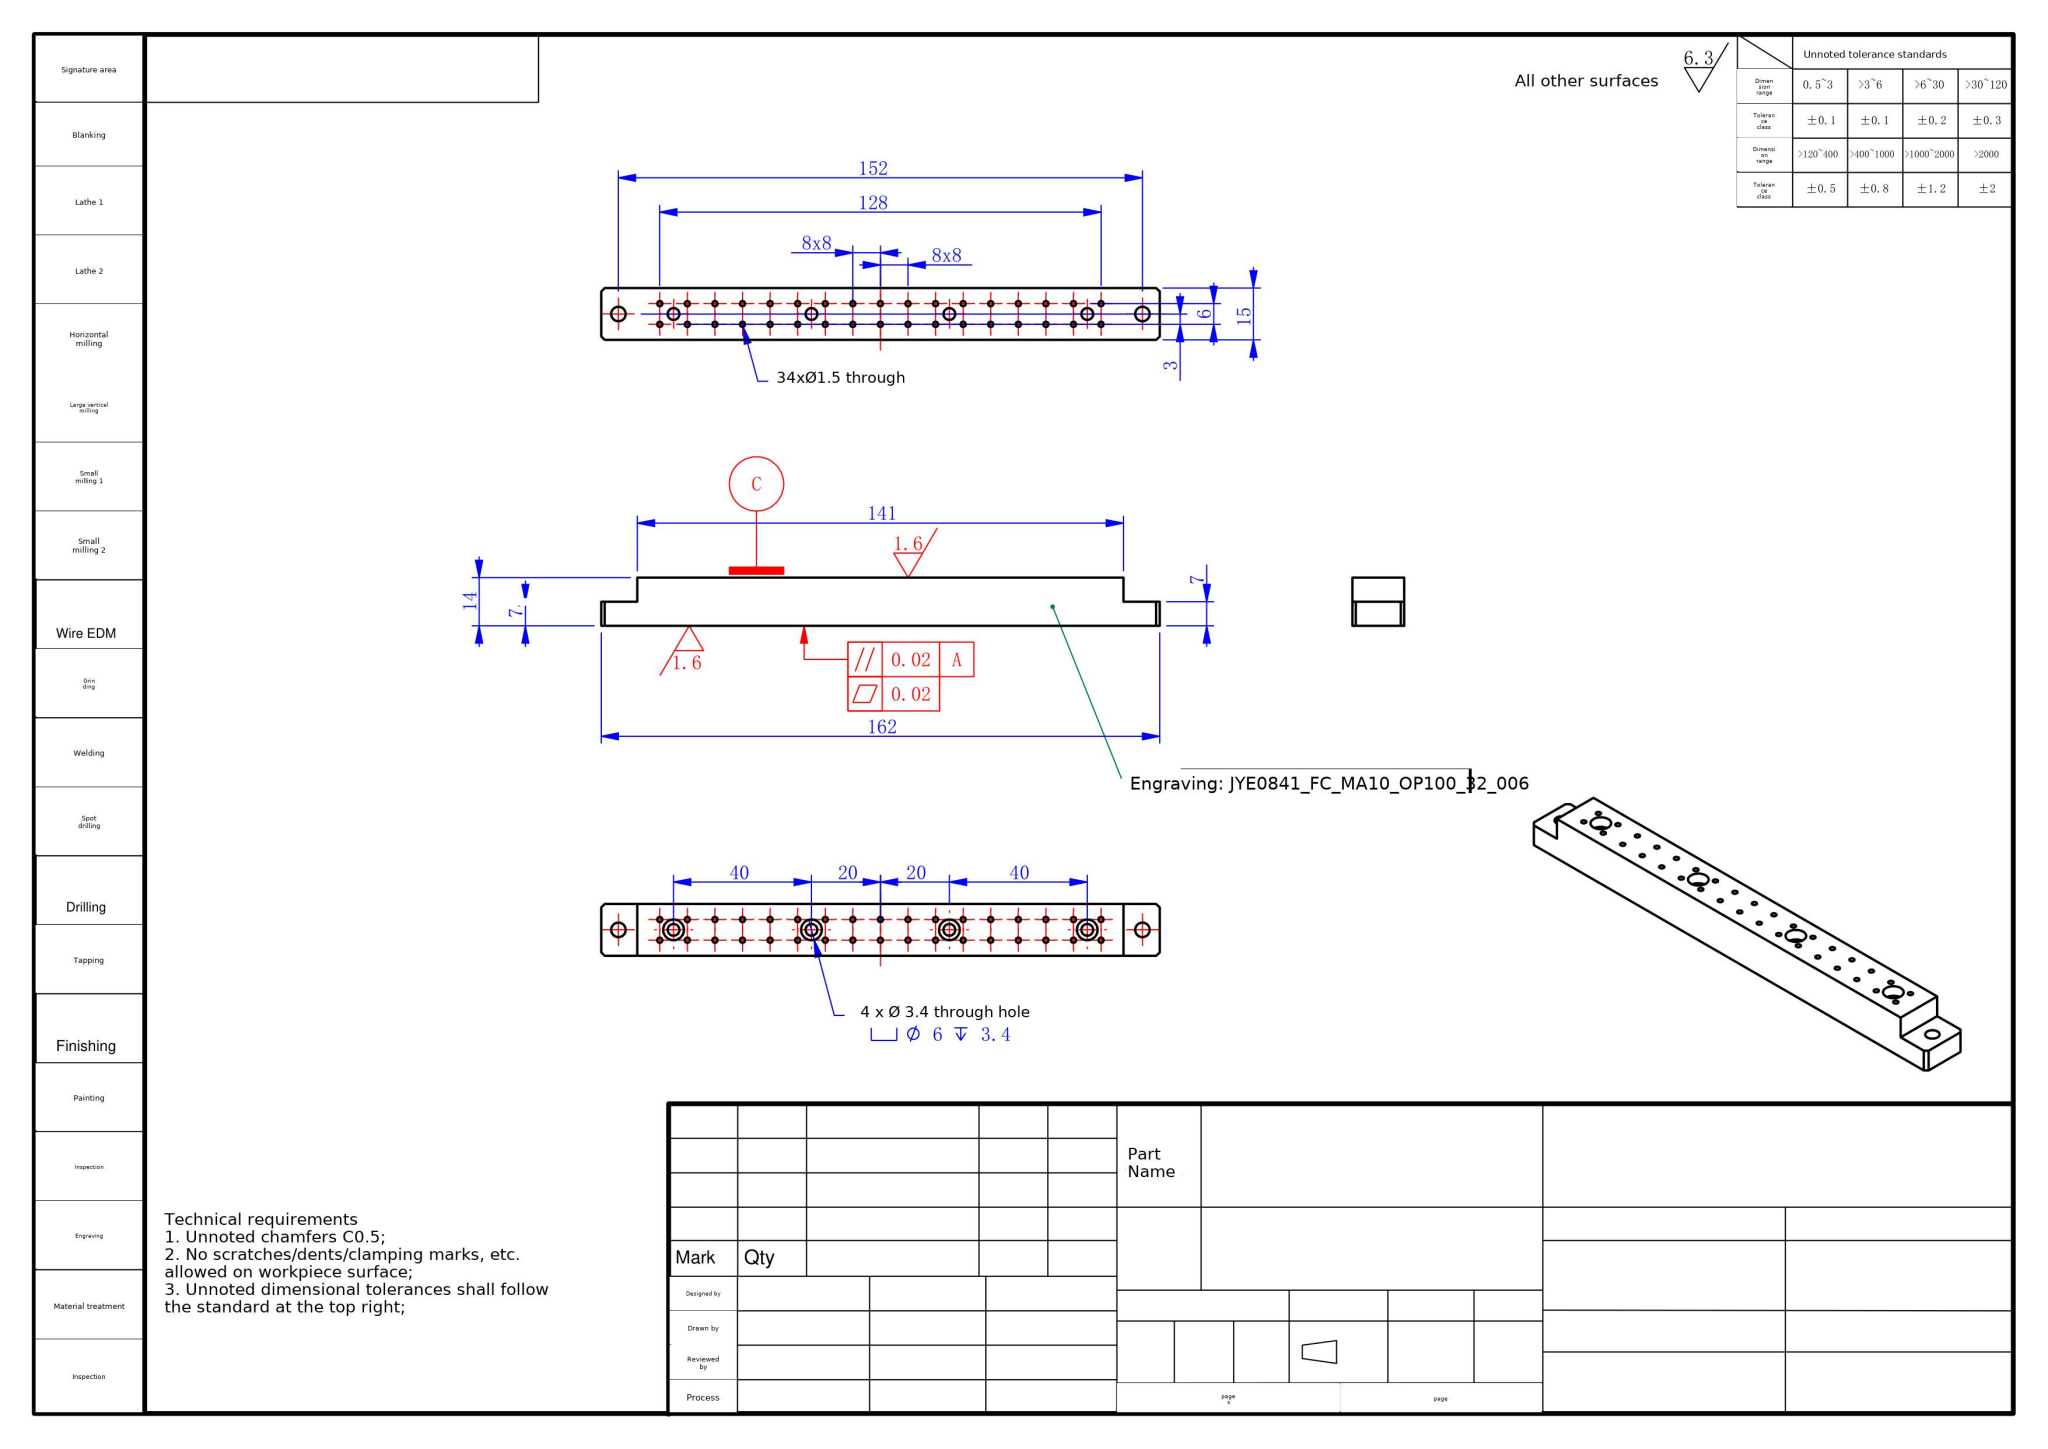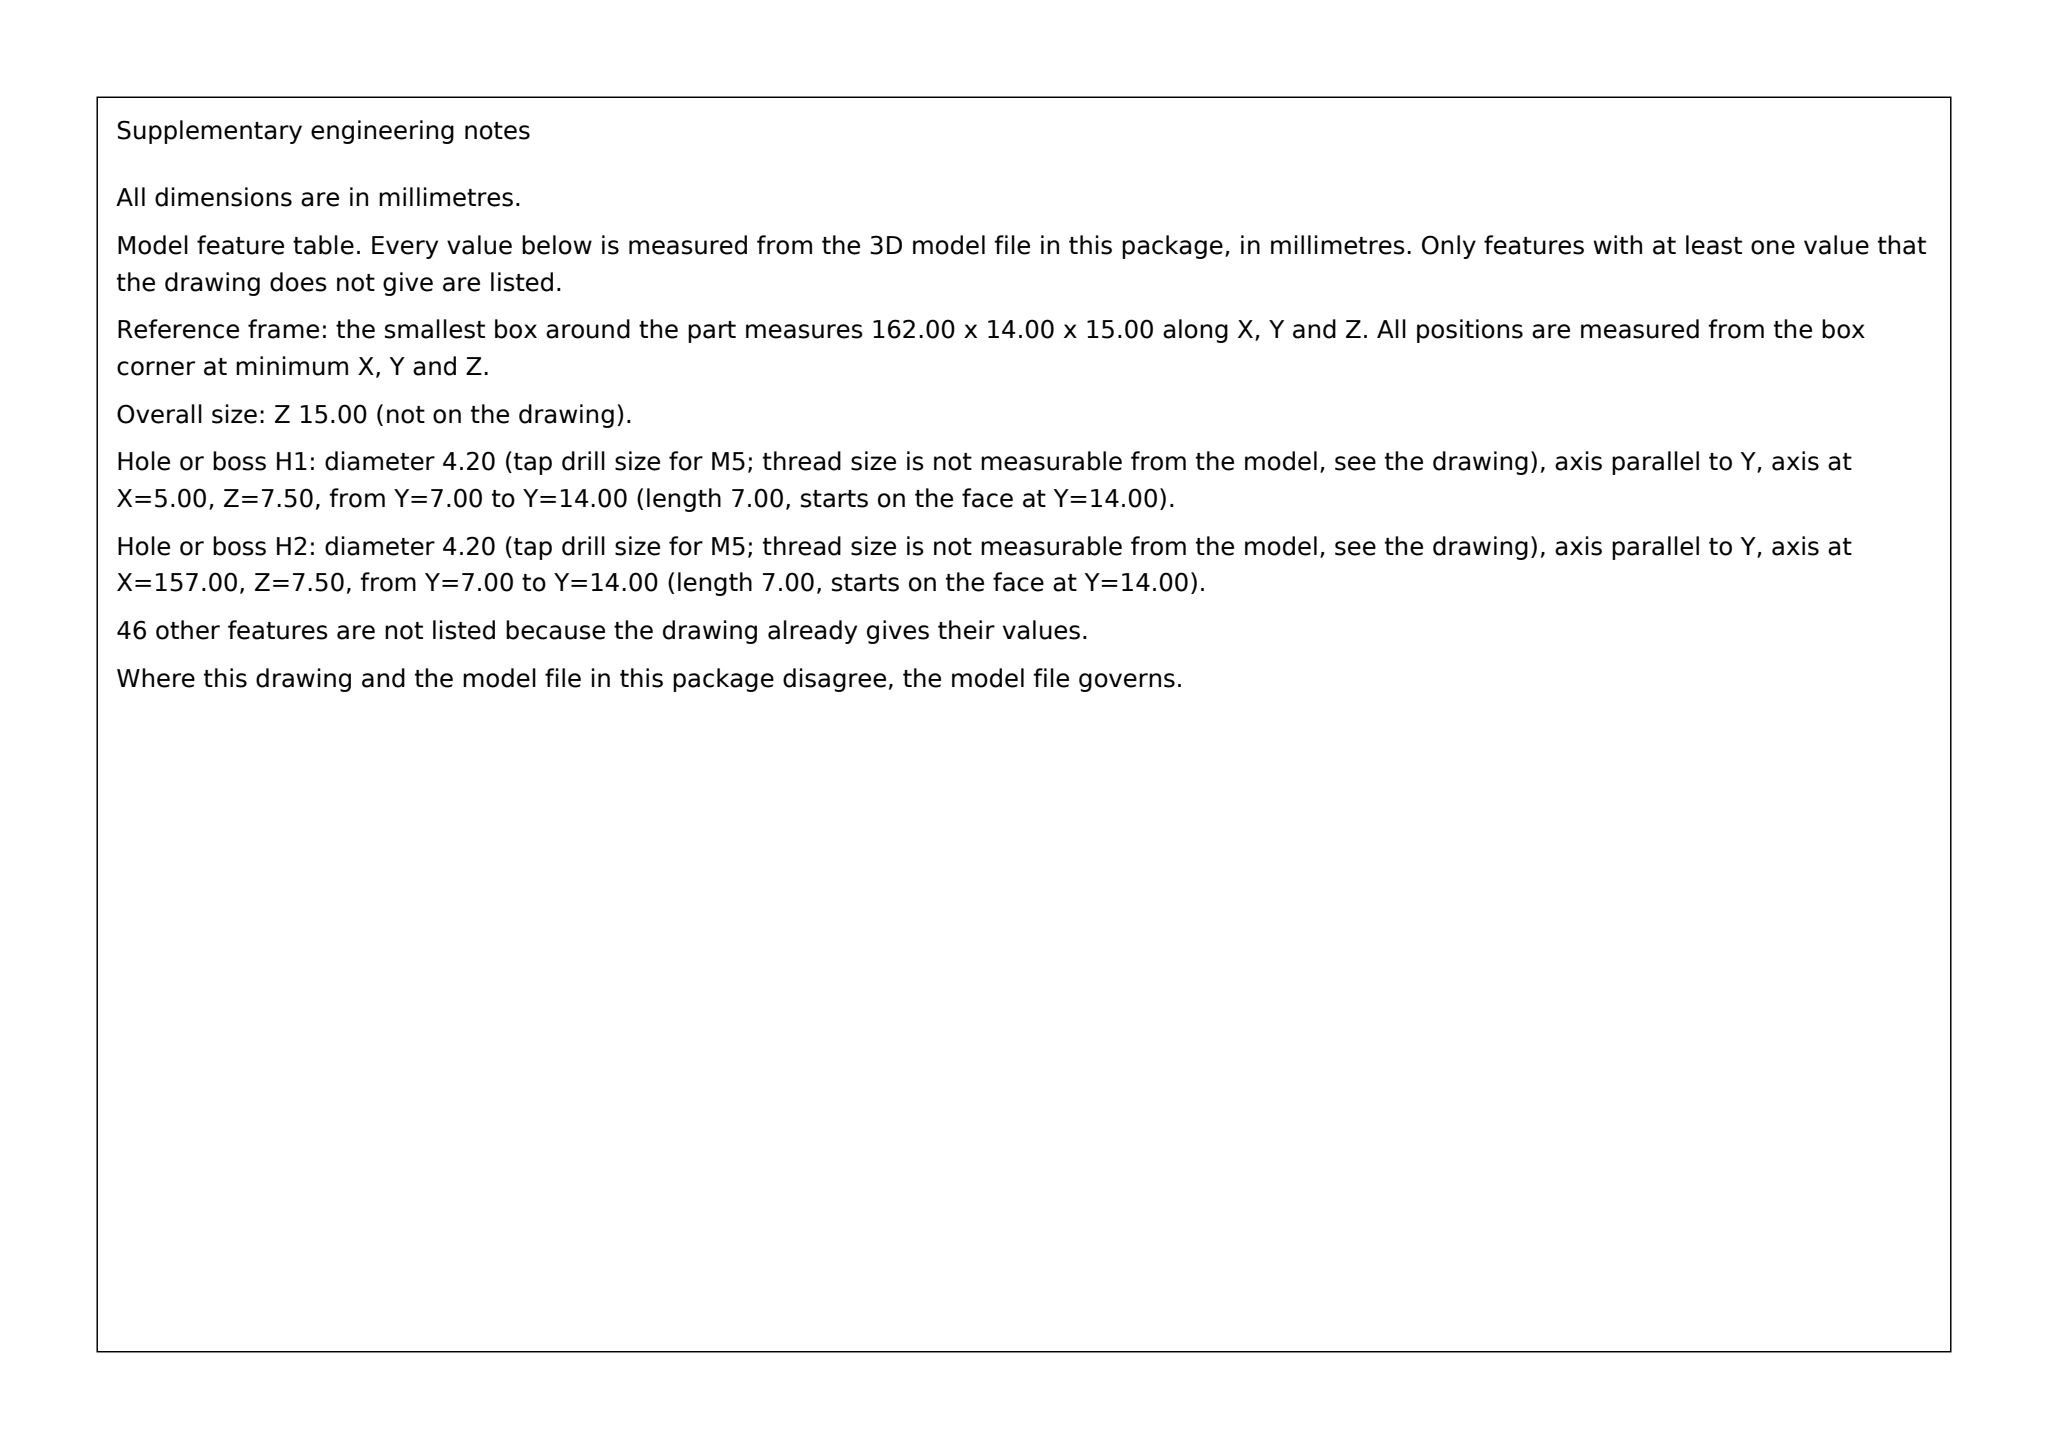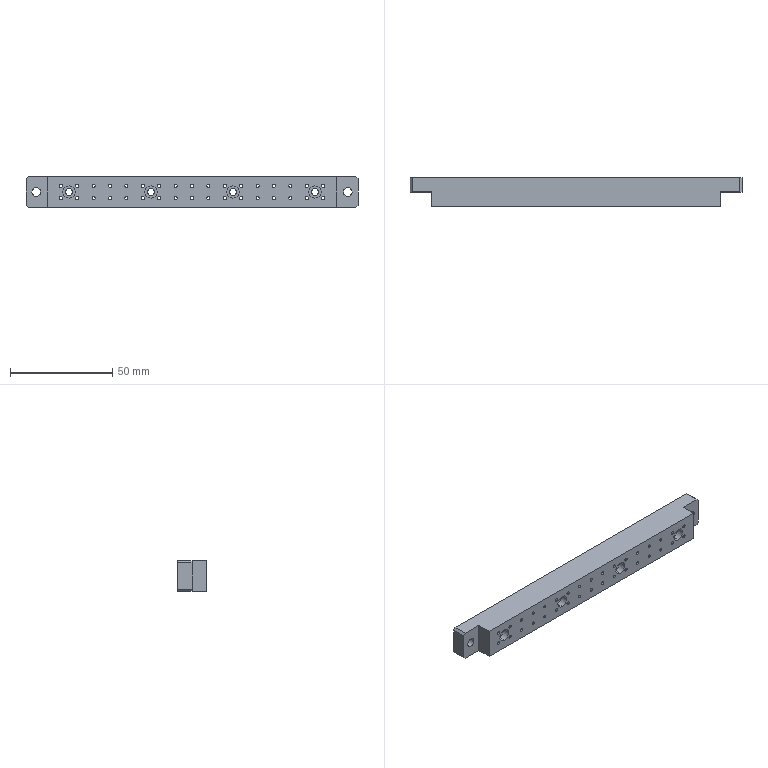Part | SolidWorks | mm | 1 solid | 106 faces | box 162 x 14 x 15 mm | volume 29996 mm3 | cylinder 88 | plane 18 | commonest cylinder face diameters 1.5 x68 6 x8 3.4 x8 4.2 x4
build123d program:
from build123d import *

# Parameters (mm, degrees)
SKETCH1_W                                         = 162
SKETCH1_H                                         = 15
BOSS_EXTRUDE1_DEPTH                               = 14
SKETCH2_W                                         = 10.5
SKETCH2_H                                         = 7
CUT_EXTRUDE1_DEPTH                                = 83.674
SKETCH3_W                                         = 10.5
SKETCH3_H                                         = 7
CUT_EXTRUDE2_DEPTH                                = 83.674
CHAMFER1_SIZE                                     = 1
HOLE_SIZE_ACCORDING_TO_TYPE_OF_HEX_SO_D           = 3.4
HOLE_SIZE_ACCORDING_TO_TYPE_OF_HEX_SO_CBORE_D     = 6
HOLE_SIZE_ACCORDING_TO_TYPE_OF_HEX_SO_CBORE_DEPTH = 3.4
SKETCH10_R                                        = 2.1
CUT_EXTRUDE3_DEPTH                                = 82.647
SKETCH11_R                                        = 0.75
CUT_EXTRUDE4_DEPTH                                = 18


with BuildPart() as part:
    # Sketch1 → Boss-Extrude1 (new body)
    with BuildSketch(Plane.XZ.offset(7)):
        Rectangle(SKETCH1_W, SKETCH1_H)
    extrude(amount=-BOSS_EXTRUDE1_DEPTH)

    # Sketch2 → Cut-Extrude1 (cut, through all)
    with BuildSketch(Plane.XY.offset(7.5)):
        with Locations((-75.75, -3.5)):
            Rectangle(SKETCH2_W, SKETCH2_H)
    extrude(amount=-CUT_EXTRUDE1_DEPTH, mode=Mode.SUBTRACT)

    # Sketch3 → Cut-Extrude2 (cut, through all)
    with BuildSketch(Plane.XY.offset(7.5)):
        with Locations((75.75, -3.5)):
            Rectangle(SKETCH3_W, SKETCH3_H)
    extrude(amount=-CUT_EXTRUDE2_DEPTH, mode=Mode.SUBTRACT)

    # Chamfer1
    chamfer1_edges = [part.edges().sort_by_distance(p)[0] for p in [
        (-81, 3.5, 7.5),
        (81, 3.5, 7.5),
        (81, 3.5, -7.5),
        (-81, 3.5, -7.5),
    ]]
    chamfer(chamfer1_edges, length=CHAMFER1_SIZE)

    # Hole Size _ according to_ Type of Hex So (through all)
    with Locations(Plane(origin=(0, -7, 0), x_dir=(-1, 0, 0), z_dir=(0, -1, 0))):
        with Locations((60, 0), (-60, 0), (-20, 0), (20, 0)):
            CounterBoreHole(HOLE_SIZE_ACCORDING_TO_TYPE_OF_HEX_SO_D / 2, HOLE_SIZE_ACCORDING_TO_TYPE_OF_HEX_SO_CBORE_D / 2, HOLE_SIZE_ACCORDING_TO_TYPE_OF_HEX_SO_CBORE_DEPTH)

    # Sketch10 → Cut-Extrude3 (cut, through all)
    with BuildSketch(Plane.XZ):
        with Locations((-76, 0)):
            Circle(SKETCH10_R)
        with Locations((76, 0)):
            Circle(SKETCH10_R)
    extrude(amount=-CUT_EXTRUDE3_DEPTH, mode=Mode.SUBTRACT)

    # Sketch11 → Cut-Extrude4 (cut)
    with BuildSketch(Plane.XZ.offset(7)):
        with Locations(Location((-8, 3, 0), (0, 0, 270))):
            Circle(SKETCH11_R)
        with Locations(Location((-8, -3, 0), (0, 0, 270))):
            Circle(SKETCH11_R)
        with Locations(Location((0, 3, 0), (0, 0, 270))):
            Circle(SKETCH11_R)
        with Locations(Location((0, -3, 0), (0, 0, 270))):
            Circle(SKETCH11_R)
        with Locations(Location((8, -3, 0), (0, 0, 270))):
            Circle(SKETCH11_R)
        with Locations(Location((8, 3, 0), (0, 0, 270))):
            Circle(SKETCH11_R)
        with Locations(Location((16, 3, 0), (0, 0, 270))):
            Circle(SKETCH11_R)
        with Locations(Location((16, -3, 0), (0, 0, 270))):
            Circle(SKETCH11_R)
        with Locations(Location((24, 3, 0), (0, 0, 270))):
            Circle(SKETCH11_R)
        with Locations(Location((24, -3, 0), (0, 0, 270))):
            Circle(SKETCH11_R)
        with Locations(Location((32, -3, 0), (0, 0, 270))):
            Circle(SKETCH11_R)
        with Locations(Location((32, 3, 0), (0, 0, 270))):
            Circle(SKETCH11_R)
        with Locations(Location((40, -3, 0), (0, 0, 270))):
            Circle(SKETCH11_R)
        with Locations(Location((40, 3, 0), (0, 0, 270))):
            Circle(SKETCH11_R)
        with Locations(Location((48, -3, 0), (0, 0, 270))):
            Circle(SKETCH11_R)
        with Locations(Location((48, 3, 0), (0, 0, 270))):
            Circle(SKETCH11_R)
        with Locations(Location((56, -3, 0), (0, 0, 270))):
            Circle(SKETCH11_R)
        with Locations(Location((56, 3, 0), (0, 0, 270))):
            Circle(SKETCH11_R)
        with Locations(Location((64, -3, 0), (0, 0, 270))):
            Circle(SKETCH11_R)
        with Locations(Location((64, 3, 0), (0, 0, 270))):
            Circle(SKETCH11_R)
        with Locations(Location((-64, 3, 0), (0, 0, 270))):
            Circle(SKETCH11_R)
        with Locations(Location((-64, -3, 0), (0, 0, 270))):
            Circle(SKETCH11_R)
        with Locations(Location((-56, 3, 0), (0, 0, 270))):
            Circle(SKETCH11_R)
        with Locations(Location((-56, -3, 0), (0, 0, 270))):
            Circle(SKETCH11_R)
        with Locations(Location((-48, 3, 0), (0, 0, 270))):
            Circle(SKETCH11_R)
        with Locations(Location((-48, -3, 0), (0, 0, 270))):
            Circle(SKETCH11_R)
        with Locations(Location((-40, 3, 0), (0, 0, 270))):
            Circle(SKETCH11_R)
        with Locations(Location((-40, -3, 0), (0, 0, 270))):
            Circle(SKETCH11_R)
        with Locations(Location((-32, 3, 0), (0, 0, 270))):
            Circle(SKETCH11_R)
        with Locations(Location((-32, -3, 0), (0, 0, 270))):
            Circle(SKETCH11_R)
        with Locations(Location((-24, -3, 0), (0, 0, 270))):
            Circle(SKETCH11_R)
        with Locations(Location((-24, 3, 0), (0, 0, 270))):
            Circle(SKETCH11_R)
        with Locations(Location((-16, 3, 0), (0, 0, 270))):
            Circle(SKETCH11_R)
        with Locations(Location((-16, -3, 0), (0, 0, 270))):
            Circle(SKETCH11_R)
    extrude(amount=-CUT_EXTRUDE4_DEPTH, mode=Mode.SUBTRACT)


solid = part.part